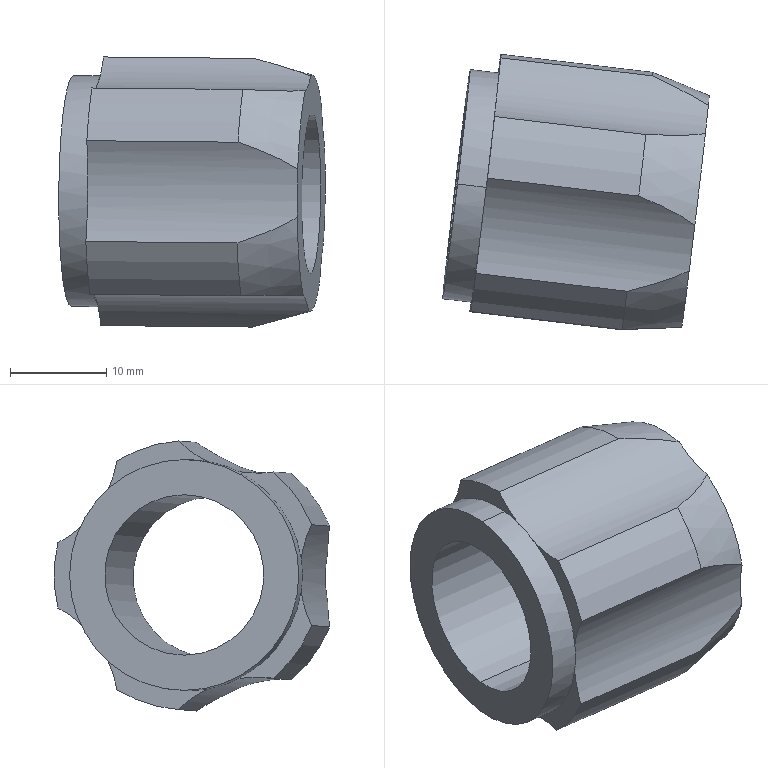Component | SolidWorks | lumu-1 | 1 solid | 33 faces | volume 7501 mm3 | cylinder 15 | plane 12 | cone 6 | commonest cylinder face diameters 23.742 x6 28 x5 16.68 x2 24 x2